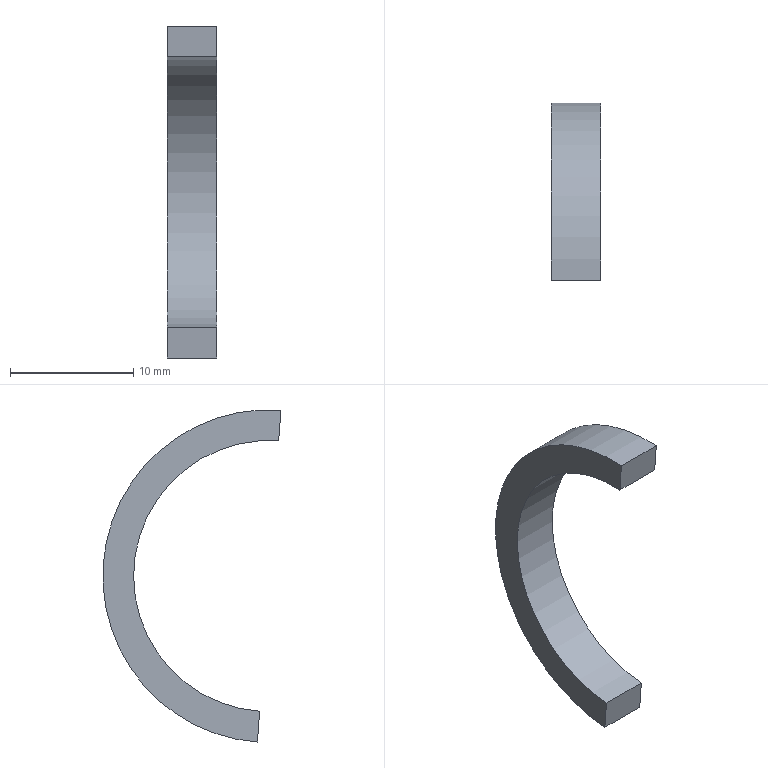Component | NX | 20C__27 | 1 solid | 6 faces | box 4 x 14.45 x 26.97 mm | volume 385 mm3 | plane 4 | cylinder 2 | commonest cylinder face diameters 22 x1 27 x1
STEP:
#1=CARTESIAN_POINT('',(0.,0.,0.));
#2=DIRECTION('',(0.,0.,1.));
#3=DIRECTION('',(1.,0.,0.));
#4=AXIS2_PLACEMENT_3D('',#1,#2,#3);
#5=CARTESIAN_POINT('',(70.022,104.66,87.007));
#6=VERTEX_POINT('',#5);
#7=CARTESIAN_POINT('',(70.022,104.836,84.514));
#8=VERTEX_POINT('',#7);
#9=CARTESIAN_POINT('',(70.022,104.66,87.007));
#10=DIRECTION('',(0.,0.07034,-0.9975));
#11=VECTOR('',#10,1.);
#12=LINE('',#9,#11);
#13=CARTESIAN_POINT('',(74.022,104.66,87.007));
#14=DIRECTION('',(0.,0.9975,0.07034));
#15=DIRECTION('',(0.,0.07034,-0.9975));
#16=AXIS2_PLACEMENT_3D('',#13,#14,#15);
#17=PLANE('',#16);
#18=CARTESIAN_POINT('',(0.,4.));
#19=DIRECTION('',(1.,0.));
#20=VECTOR('',#19,1.);
#21=LINE('',#18,#20);
#22=(GEOMETRIC_REPRESENTATION_CONTEXT(2)PARAMETRIC_REPRESENTATION_CONTEXT()REPRESENTATION_CONTEXT('',''));
#23=DEFINITIONAL_REPRESENTATION('',(#21),#22);
#24=PCURVE('',#17,#23);
#25=CARTESIAN_POINT('',(70.022,105.61,73.541));
#26=DIRECTION('',(-1.,0.,0.));
#27=DIRECTION('',(0.,0.9975,0.07034));
#28=AXIS2_PLACEMENT_3D('',#25,#26,#27);
#29=PLANE('',#28);
#30=CARTESIAN_POINT('',(-0.,-13.5));
#31=DIRECTION('',(0.,1.));
#32=VECTOR('',#31,1.);
#33=LINE('',#30,#32);
#34=(GEOMETRIC_REPRESENTATION_CONTEXT(2)PARAMETRIC_REPRESENTATION_CONTEXT()REPRESENTATION_CONTEXT('',''));
#35=DEFINITIONAL_REPRESENTATION('',(#33),#34);
#36=PCURVE('',#29,#35);
#37=SURFACE_CURVE('',#12,(#24,#36),.PCURVE_S1.);
#38=EDGE_CURVE('',#6,#8,#37,.T.);
#39=ORIENTED_EDGE('',*,*,#38,.T.);
#40=CARTESIAN_POINT('',(74.022,104.836,84.514));
#41=VERTEX_POINT('',#40);
#42=CARTESIAN_POINT('',(74.022,104.836,84.514));
#43=DIRECTION('',(-1.,0.,0.));
#44=VECTOR('',#43,1.);
#45=LINE('',#42,#44);
#46=CARTESIAN_POINT('',(2.5,0.));
#47=DIRECTION('',(0.,1.));
#48=VECTOR('',#47,1.);
#49=LINE('',#46,#48);
#50=(GEOMETRIC_REPRESENTATION_CONTEXT(2)PARAMETRIC_REPRESENTATION_CONTEXT()REPRESENTATION_CONTEXT('',''));
#51=DEFINITIONAL_REPRESENTATION('',(#49),#50);
#52=PCURVE('',#17,#51);
#53=CARTESIAN_POINT('',(74.022,105.61,73.541));
#54=DIRECTION('',(-1.,0.,0.));
#55=DIRECTION('',(0.,0.9975,0.07034));
#56=AXIS2_PLACEMENT_3D('',#53,#54,#55);
#57=CYLINDRICAL_SURFACE('',#56,11.);
#58=CARTESIAN_POINT('',(4.712,0.));
#59=DIRECTION('',(0.,1.));
#60=VECTOR('',#59,1.);
#61=LINE('',#58,#60);
#62=(GEOMETRIC_REPRESENTATION_CONTEXT(2)PARAMETRIC_REPRESENTATION_CONTEXT()REPRESENTATION_CONTEXT('',''));
#63=DEFINITIONAL_REPRESENTATION('',(#61),#62);
#64=PCURVE('',#57,#63);
#65=SURFACE_CURVE('',#45,(#52,#64),.PCURVE_S1.);
#66=EDGE_CURVE('',#41,#8,#65,.T.);
#67=ORIENTED_EDGE('',*,*,#66,.F.);
#68=CARTESIAN_POINT('',(74.022,104.66,87.007));
#69=VERTEX_POINT('',#68);
#70=CARTESIAN_POINT('',(74.022,104.66,87.007));
#71=DIRECTION('',(0.,0.07034,-0.9975));
#72=VECTOR('',#71,1.);
#73=LINE('',#70,#72);
#74=CARTESIAN_POINT('',(0.,0.));
#75=DIRECTION('',(1.,0.));
#76=VECTOR('',#75,1.);
#77=LINE('',#74,#76);
#78=(GEOMETRIC_REPRESENTATION_CONTEXT(2)PARAMETRIC_REPRESENTATION_CONTEXT()REPRESENTATION_CONTEXT('',''));
#79=DEFINITIONAL_REPRESENTATION('',(#77),#78);
#80=PCURVE('',#17,#79);
#81=CARTESIAN_POINT('',(74.022,105.61,73.541));
#82=DIRECTION('',(-1.,0.,0.));
#83=DIRECTION('',(0.,0.9975,0.07034));
#84=AXIS2_PLACEMENT_3D('',#81,#82,#83);
#85=PLANE('',#84);
#86=CARTESIAN_POINT('',(-0.,-13.5));
#87=DIRECTION('',(0.,1.));
#88=VECTOR('',#87,1.);
#89=LINE('',#86,#88);
#90=(GEOMETRIC_REPRESENTATION_CONTEXT(2)PARAMETRIC_REPRESENTATION_CONTEXT()REPRESENTATION_CONTEXT('',''));
#91=DEFINITIONAL_REPRESENTATION('',(#89),#90);
#92=PCURVE('',#85,#91);
#93=SURFACE_CURVE('',#73,(#80,#92),.PCURVE_S1.);
#94=EDGE_CURVE('',#69,#41,#93,.T.);
#95=ORIENTED_EDGE('',*,*,#94,.F.);
#96=CARTESIAN_POINT('',(74.022,104.66,87.007));
#97=DIRECTION('',(-1.,0.,0.));
#98=VECTOR('',#97,1.);
#99=LINE('',#96,#98);
#100=CARTESIAN_POINT('',(0.,0.));
#101=DIRECTION('',(0.,1.));
#102=VECTOR('',#101,1.);
#103=LINE('',#100,#102);
#104=(GEOMETRIC_REPRESENTATION_CONTEXT(2)PARAMETRIC_REPRESENTATION_CONTEXT()REPRESENTATION_CONTEXT('',''));
#105=DEFINITIONAL_REPRESENTATION('',(#103),#104);
#106=PCURVE('',#17,#105);
#107=CARTESIAN_POINT('',(74.022,105.61,73.541));
#108=DIRECTION('',(-1.,0.,0.));
#109=DIRECTION('',(0.,0.9975,0.07034));
#110=AXIS2_PLACEMENT_3D('',#107,#108,#109);
#111=CYLINDRICAL_SURFACE('',#110,13.5);
#112=CARTESIAN_POINT('',(4.712,0.));
#113=DIRECTION('',(0.,1.));
#114=VECTOR('',#113,1.);
#115=LINE('',#112,#114);
#116=(GEOMETRIC_REPRESENTATION_CONTEXT(2)PARAMETRIC_REPRESENTATION_CONTEXT()REPRESENTATION_CONTEXT('',''));
#117=DEFINITIONAL_REPRESENTATION('',(#115),#116);
#118=PCURVE('',#111,#117);
#119=SURFACE_CURVE('',#99,(#106,#118),.PCURVE_S1.);
#120=EDGE_CURVE('',#69,#6,#119,.T.);
#121=ORIENTED_EDGE('',*,*,#120,.T.);
#122=EDGE_LOOP('',(#39,#67,#95,#121));
#123=FACE_BOUND('',#122,.T.);
#124=ADVANCED_FACE('',(#123),#17,.F.);
#125=ORIENTED_EDGE('',*,*,#66,.F.);
#126=CARTESIAN_POINT('',(74.022,106.383,62.568));
#127=VERTEX_POINT('',#126);
#128=CARTESIAN_POINT('',(74.022,105.61,73.541));
#129=DIRECTION('',(-1.,0.,0.));
#130=DIRECTION('',(0.,0.07034,-0.9975));
#131=AXIS2_PLACEMENT_3D('',#128,#129,#130);
#132=CIRCLE('',#131,11.);
#133=CARTESIAN_POINT('',(1.571,0.));
#134=DIRECTION('',(1.,0.));
#135=VECTOR('',#134,1.);
#136=LINE('',#133,#135);
#137=(GEOMETRIC_REPRESENTATION_CONTEXT(2)PARAMETRIC_REPRESENTATION_CONTEXT()REPRESENTATION_CONTEXT('',''));
#138=DEFINITIONAL_REPRESENTATION('',(#136),#137);
#139=PCURVE('',#57,#138);
#140=CARTESIAN_POINT('',(0.,0.));
#141=DIRECTION('',(-0.,1.));
#142=AXIS2_PLACEMENT_2D('',#140,#141);
#143=CIRCLE('',#142,11.);
#144=(GEOMETRIC_REPRESENTATION_CONTEXT(2)PARAMETRIC_REPRESENTATION_CONTEXT()REPRESENTATION_CONTEXT('',''));
#145=DEFINITIONAL_REPRESENTATION('',(#143),#144);
#146=PCURVE('',#85,#145);
#147=SURFACE_CURVE('',#132,(#139,#146),.PCURVE_S1.);
#148=EDGE_CURVE('',#41,#127,#147,.T.);
#149=ORIENTED_EDGE('',*,*,#148,.T.);
#150=CARTESIAN_POINT('',(70.022,106.383,62.568));
#151=VERTEX_POINT('',#150);
#152=CARTESIAN_POINT('',(74.022,106.383,62.568));
#153=DIRECTION('',(-1.,0.,0.));
#154=VECTOR('',#153,1.);
#155=LINE('',#152,#154);
#156=CARTESIAN_POINT('',(7.854,0.));
#157=DIRECTION('',(0.,1.));
#158=VECTOR('',#157,1.);
#159=LINE('',#156,#158);
#160=(GEOMETRIC_REPRESENTATION_CONTEXT(2)PARAMETRIC_REPRESENTATION_CONTEXT()REPRESENTATION_CONTEXT('',''));
#161=DEFINITIONAL_REPRESENTATION('',(#159),#160);
#162=PCURVE('',#57,#161);
#163=CARTESIAN_POINT('',(74.022,106.383,62.568));
#164=DIRECTION('',(0.,0.9975,0.07034));
#165=DIRECTION('',(0.,0.07034,-0.9975));
#166=AXIS2_PLACEMENT_3D('',#163,#164,#165);
#167=PLANE('',#166);
#168=CARTESIAN_POINT('',(0.,0.));
#169=DIRECTION('',(0.,1.));
#170=VECTOR('',#169,1.);
#171=LINE('',#168,#170);
#172=(GEOMETRIC_REPRESENTATION_CONTEXT(2)PARAMETRIC_REPRESENTATION_CONTEXT()REPRESENTATION_CONTEXT('',''));
#173=DEFINITIONAL_REPRESENTATION('',(#171),#172);
#174=PCURVE('',#167,#173);
#175=SURFACE_CURVE('',#155,(#162,#174),.PCURVE_S1.);
#176=EDGE_CURVE('',#127,#151,#175,.T.);
#177=ORIENTED_EDGE('',*,*,#176,.T.);
#178=CARTESIAN_POINT('',(70.022,105.61,73.541));
#179=DIRECTION('',(-1.,0.,0.));
#180=DIRECTION('',(0.,0.07034,-0.9975));
#181=AXIS2_PLACEMENT_3D('',#178,#179,#180);
#182=CIRCLE('',#181,11.);
#183=CARTESIAN_POINT('',(1.571,4.));
#184=DIRECTION('',(1.,0.));
#185=VECTOR('',#184,1.);
#186=LINE('',#183,#185);
#187=(GEOMETRIC_REPRESENTATION_CONTEXT(2)PARAMETRIC_REPRESENTATION_CONTEXT()REPRESENTATION_CONTEXT('',''));
#188=DEFINITIONAL_REPRESENTATION('',(#186),#187);
#189=PCURVE('',#57,#188);
#190=CARTESIAN_POINT('',(0.,0.));
#191=DIRECTION('',(-0.,1.));
#192=AXIS2_PLACEMENT_2D('',#190,#191);
#193=CIRCLE('',#192,11.);
#194=(GEOMETRIC_REPRESENTATION_CONTEXT(2)PARAMETRIC_REPRESENTATION_CONTEXT()REPRESENTATION_CONTEXT('',''));
#195=DEFINITIONAL_REPRESENTATION('',(#193),#194);
#196=PCURVE('',#29,#195);
#197=SURFACE_CURVE('',#182,(#189,#196),.PCURVE_S1.);
#198=EDGE_CURVE('',#8,#151,#197,.T.);
#199=ORIENTED_EDGE('',*,*,#198,.F.);
#200=EDGE_LOOP('',(#125,#149,#177,#199));
#201=FACE_BOUND('',#200,.F.);
#202=ADVANCED_FACE('',(#201),#57,.F.);
#203=CARTESIAN_POINT('',(70.022,106.559,60.074));
#204=VERTEX_POINT('',#203);
#205=CARTESIAN_POINT('',(70.022,106.383,62.568));
#206=DIRECTION('',(0.,0.07034,-0.9975));
#207=VECTOR('',#206,1.);
#208=LINE('',#205,#207);
#209=CARTESIAN_POINT('',(0.,4.));
#210=DIRECTION('',(1.,0.));
#211=VECTOR('',#210,1.);
#212=LINE('',#209,#211);
#213=(GEOMETRIC_REPRESENTATION_CONTEXT(2)PARAMETRIC_REPRESENTATION_CONTEXT()REPRESENTATION_CONTEXT('',''));
#214=DEFINITIONAL_REPRESENTATION('',(#212),#213);
#215=PCURVE('',#167,#214);
#216=CARTESIAN_POINT('',(0.,11.));
#217=DIRECTION('',(0.,1.));
#218=VECTOR('',#217,1.);
#219=LINE('',#216,#218);
#220=(GEOMETRIC_REPRESENTATION_CONTEXT(2)PARAMETRIC_REPRESENTATION_CONTEXT()REPRESENTATION_CONTEXT('',''));
#221=DEFINITIONAL_REPRESENTATION('',(#219),#220);
#222=PCURVE('',#29,#221);
#223=SURFACE_CURVE('',#208,(#215,#222),.PCURVE_S1.);
#224=EDGE_CURVE('',#151,#204,#223,.T.);
#225=ORIENTED_EDGE('',*,*,#224,.T.);
#226=CARTESIAN_POINT('',(74.022,106.559,60.074));
#227=VERTEX_POINT('',#226);
#228=CARTESIAN_POINT('',(74.022,106.559,60.074));
#229=DIRECTION('',(-1.,0.,0.));
#230=VECTOR('',#229,1.);
#231=LINE('',#228,#230);
#232=CARTESIAN_POINT('',(2.5,0.));
#233=DIRECTION('',(0.,1.));
#234=VECTOR('',#233,1.);
#235=LINE('',#232,#234);
#236=(GEOMETRIC_REPRESENTATION_CONTEXT(2)PARAMETRIC_REPRESENTATION_CONTEXT()REPRESENTATION_CONTEXT('',''));
#237=DEFINITIONAL_REPRESENTATION('',(#235),#236);
#238=PCURVE('',#167,#237);
#239=CARTESIAN_POINT('',(7.854,0.));
#240=DIRECTION('',(0.,1.));
#241=VECTOR('',#240,1.);
#242=LINE('',#239,#241);
#243=(GEOMETRIC_REPRESENTATION_CONTEXT(2)PARAMETRIC_REPRESENTATION_CONTEXT()REPRESENTATION_CONTEXT('',''));
#244=DEFINITIONAL_REPRESENTATION('',(#242),#243);
#245=PCURVE('',#111,#244);
#246=SURFACE_CURVE('',#231,(#238,#245),.PCURVE_S1.);
#247=EDGE_CURVE('',#227,#204,#246,.T.);
#248=ORIENTED_EDGE('',*,*,#247,.F.);
#249=CARTESIAN_POINT('',(74.022,106.383,62.568));
#250=DIRECTION('',(0.,0.07034,-0.9975));
#251=VECTOR('',#250,1.);
#252=LINE('',#249,#251);
#253=CARTESIAN_POINT('',(0.,0.));
#254=DIRECTION('',(1.,0.));
#255=VECTOR('',#254,1.);
#256=LINE('',#253,#255);
#257=(GEOMETRIC_REPRESENTATION_CONTEXT(2)PARAMETRIC_REPRESENTATION_CONTEXT()REPRESENTATION_CONTEXT('',''));
#258=DEFINITIONAL_REPRESENTATION('',(#256),#257);
#259=PCURVE('',#167,#258);
#260=CARTESIAN_POINT('',(0.,11.));
#261=DIRECTION('',(0.,1.));
#262=VECTOR('',#261,1.);
#263=LINE('',#260,#262);
#264=(GEOMETRIC_REPRESENTATION_CONTEXT(2)PARAMETRIC_REPRESENTATION_CONTEXT()REPRESENTATION_CONTEXT('',''));
#265=DEFINITIONAL_REPRESENTATION('',(#263),#264);
#266=PCURVE('',#85,#265);
#267=SURFACE_CURVE('',#252,(#259,#266),.PCURVE_S1.);
#268=EDGE_CURVE('',#127,#227,#267,.T.);
#269=ORIENTED_EDGE('',*,*,#268,.F.);
#270=ORIENTED_EDGE('',*,*,#176,.T.);
#271=EDGE_LOOP('',(#225,#248,#269,#270));
#272=FACE_BOUND('',#271,.T.);
#273=ADVANCED_FACE('',(#272),#167,.F.);
#274=CARTESIAN_POINT('',(70.022,105.61,73.541));
#275=DIRECTION('',(1.,0.,0.));
#276=DIRECTION('',(0.,0.07034,-0.9975));
#277=AXIS2_PLACEMENT_3D('',#274,#275,#276);
#278=CIRCLE('',#277,13.5);
#279=CARTESIAN_POINT('',(7.854,4.));
#280=DIRECTION('',(-1.,0.));
#281=VECTOR('',#280,1.);
#282=LINE('',#279,#281);
#283=(GEOMETRIC_REPRESENTATION_CONTEXT(2)PARAMETRIC_REPRESENTATION_CONTEXT()REPRESENTATION_CONTEXT('',''));
#284=DEFINITIONAL_REPRESENTATION('',(#282),#283);
#285=PCURVE('',#111,#284);
#286=CARTESIAN_POINT('',(0.,13.5));
#287=CARTESIAN_POINT('',(23.383,13.5));
#288=CARTESIAN_POINT('',(11.691,-6.75));
#289=CARTESIAN_POINT('',(-0.,-27.));
#290=CARTESIAN_POINT('',(-11.691,-6.75));
#291=CARTESIAN_POINT('',(-23.383,13.5));
#292=CARTESIAN_POINT('',(0.,13.5));
#293=(BOUNDED_CURVE()B_SPLINE_CURVE(2,(#286,#287,#288,#289,#290,#291,#292),.UNSPECIFIED.,.T.,.F.)B_SPLINE_CURVE_WITH_KNOTS((1,2,2,2,2,1),(-2.094,0.,2.094,4.189,6.283,8.378),.UNSPECIFIED.)CURVE()GEOMETRIC_REPRESENTATION_ITEM()RATIONAL_B_SPLINE_CURVE((1.,0.5,1.,0.5,1.,0.5,1.))REPRESENTATION_ITEM(''));
#294=(GEOMETRIC_REPRESENTATION_CONTEXT(2)PARAMETRIC_REPRESENTATION_CONTEXT()REPRESENTATION_CONTEXT('',''));
#295=DEFINITIONAL_REPRESENTATION('',(#293),#294);
#296=PCURVE('',#29,#295);
#297=SURFACE_CURVE('',#278,(#285,#296),.PCURVE_S1.);
#298=EDGE_CURVE('',#204,#6,#297,.T.);
#299=ORIENTED_EDGE('',*,*,#298,.T.);
#300=ORIENTED_EDGE('',*,*,#120,.F.);
#301=CARTESIAN_POINT('',(74.022,105.61,73.541));
#302=DIRECTION('',(1.,0.,0.));
#303=DIRECTION('',(0.,0.07034,-0.9975));
#304=AXIS2_PLACEMENT_3D('',#301,#302,#303);
#305=CIRCLE('',#304,13.5);
#306=CARTESIAN_POINT('',(7.854,0.));
#307=DIRECTION('',(-1.,0.));
#308=VECTOR('',#307,1.);
#309=LINE('',#306,#308);
#310=(GEOMETRIC_REPRESENTATION_CONTEXT(2)PARAMETRIC_REPRESENTATION_CONTEXT()REPRESENTATION_CONTEXT('',''));
#311=DEFINITIONAL_REPRESENTATION('',(#309),#310);
#312=PCURVE('',#111,#311);
#313=CARTESIAN_POINT('',(0.,13.5));
#314=CARTESIAN_POINT('',(23.383,13.5));
#315=CARTESIAN_POINT('',(11.691,-6.75));
#316=CARTESIAN_POINT('',(-0.,-27.));
#317=CARTESIAN_POINT('',(-11.691,-6.75));
#318=CARTESIAN_POINT('',(-23.383,13.5));
#319=CARTESIAN_POINT('',(0.,13.5));
#320=(BOUNDED_CURVE()B_SPLINE_CURVE(2,(#313,#314,#315,#316,#317,#318,#319),.UNSPECIFIED.,.T.,.F.)B_SPLINE_CURVE_WITH_KNOTS((1,2,2,2,2,1),(-2.094,0.,2.094,4.189,6.283,8.378),.UNSPECIFIED.)CURVE()GEOMETRIC_REPRESENTATION_ITEM()RATIONAL_B_SPLINE_CURVE((1.,0.5,1.,0.5,1.,0.5,1.))REPRESENTATION_ITEM(''));
#321=(GEOMETRIC_REPRESENTATION_CONTEXT(2)PARAMETRIC_REPRESENTATION_CONTEXT()REPRESENTATION_CONTEXT('',''));
#322=DEFINITIONAL_REPRESENTATION('',(#320),#321);
#323=PCURVE('',#85,#322);
#324=SURFACE_CURVE('',#305,(#312,#323),.PCURVE_S1.);
#325=EDGE_CURVE('',#227,#69,#324,.T.);
#326=ORIENTED_EDGE('',*,*,#325,.F.);
#327=ORIENTED_EDGE('',*,*,#247,.T.);
#328=EDGE_LOOP('',(#299,#300,#326,#327));
#329=FACE_BOUND('',#328,.T.);
#330=ADVANCED_FACE('',(#329),#111,.T.);
#331=ORIENTED_EDGE('',*,*,#94,.T.);
#332=ORIENTED_EDGE('',*,*,#148,.T.);
#333=ORIENTED_EDGE('',*,*,#268,.T.);
#334=ORIENTED_EDGE('',*,*,#325,.T.);
#335=EDGE_LOOP('',(#331,#332,#333,#334));
#336=FACE_BOUND('',#335,.T.);
#337=ADVANCED_FACE('',(#336),#85,.F.);
#338=ORIENTED_EDGE('',*,*,#38,.F.);
#339=ORIENTED_EDGE('',*,*,#298,.F.);
#340=ORIENTED_EDGE('',*,*,#224,.F.);
#341=ORIENTED_EDGE('',*,*,#198,.F.);
#342=EDGE_LOOP('',(#338,#339,#340,#341));
#343=FACE_BOUND('',#342,.T.);
#344=ADVANCED_FACE('',(#343),#29,.T.);
#345=CLOSED_SHELL('',(#124,#202,#273,#330,#337,#344));
#346=MANIFOLD_SOLID_BREP('',#345);
#347=(LENGTH_UNIT()NAMED_UNIT(*)SI_UNIT(.MILLI.,.METRE.));
#348=UNCERTAINTY_MEASURE_WITH_UNIT(LENGTH_MEASURE(0.0000001),#347,'','');
#349=(NAMED_UNIT(*)PLANE_ANGLE_UNIT()SI_UNIT($,.RADIAN.));
#350=(NAMED_UNIT(*)SI_UNIT($,.STERADIAN.)SOLID_ANGLE_UNIT());
#351=(GEOMETRIC_REPRESENTATION_CONTEXT(3)GLOBAL_UNCERTAINTY_ASSIGNED_CONTEXT((#348))GLOBAL_UNIT_ASSIGNED_CONTEXT((#347,#349,#350))REPRESENTATION_CONTEXT('',''));
#352=ADVANCED_BREP_SHAPE_REPRESENTATION('',(#4,#346),#351);